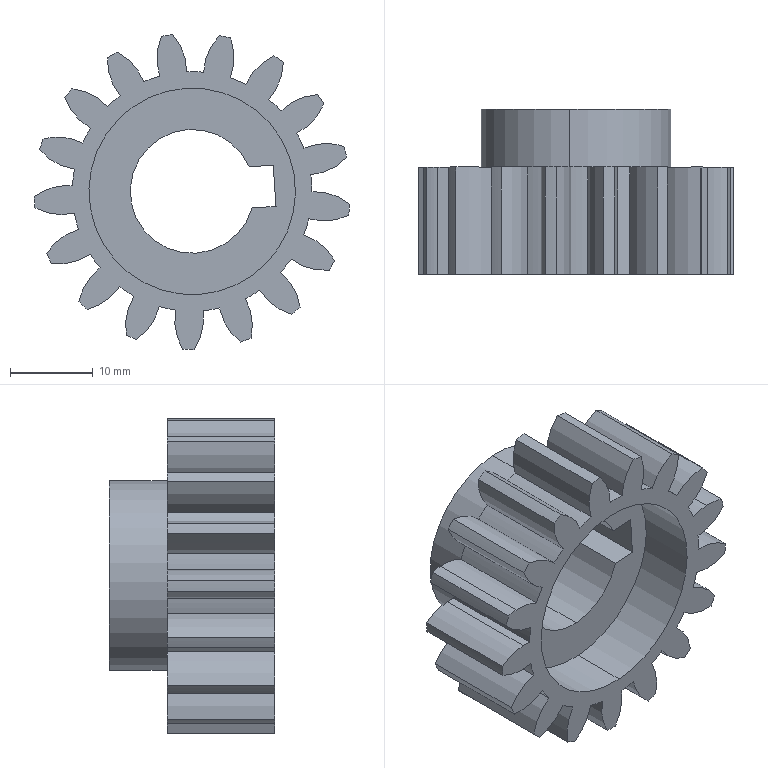Component | SolidWorks | GenevaWheelUpperGear(45Steel)-1 | 1 solid | 86 faces | box 38.22 x 20 x 38.14 mm | volume 8625 mm3 | cylinder 79 | plane 7 | commonest cylinder face diameters 13.6 x38 29 x17 38.289 x17 15 x3 25 x2 23 x2
build123d program:
from build123d import *

# Parameters (mm, degrees)
SKETCH1_R           = 14.5
BOSS_EXTRUDE1_DEPTH = 20
BOSS_EXTRUDE2_START = -13
BOSS_EXTRUDE2_DEPTH = 13
SKETCH4_R           = 14.5
SKETCH4_R_2         = 11.5
CUT_EXTRUDE1_DEPTH  = 7
CIRPATTERN1_COUNT   = 17
SKETCH5_R           = 12.5
CUT_EXTRUDE2_DEPTH  = 7


with BuildPart() as part:
    # Sketch1 → Boss-Extrude1 (new body)
    with BuildSketch(Plane.XY):
        Circle(SKETCH1_R)
        with BuildLine():
            Line((-2.5, -10), (2.5, -10))
            Line((2.5, -10), (2.5, -7.071))
            ThreePointArc((2.5, -7.071), (0, 7.5), (-2.5, -7.071))
            Line((-2.5, -7.071), (-2.5, -10))
        make_face(mode=Mode.SUBTRACT)
    extrude(amount=BOSS_EXTRUDE1_DEPTH)

    # Sketch3 → Boss-Extrude2 (add)
    with BuildSketch(Plane.XY.offset(20).offset(BOSS_EXTRUDE2_START)):
        with BuildLine():
            ThreePointArc((0.6859, 19.132), (0, 19.144), (-0.6859, 19.132))
            ThreePointArc((-0.6859, 19.132), (-1.604, 16.857), (-1.655, 14.405))
            ThreePointArc((-1.655, 14.405), (0, 14.5), (1.655, 14.405))
            ThreePointArc((1.655, 14.405), (1.604, 16.857), (0.6859, 19.132))
        make_face()
    boss_extrude2 = extrude(amount=BOSS_EXTRUDE2_DEPTH)

    # Sketch4 → Cut-Extrude1 (cut)
    with BuildSketch(Plane(origin=(0, 0, 0), x_dir=(-1, 0, 0), z_dir=(0, 0, -1))):
        Circle(SKETCH4_R)
        Circle(SKETCH4_R_2, mode=Mode.SUBTRACT)
    extrude(amount=-CUT_EXTRUDE1_DEPTH, mode=Mode.SUBTRACT)

    # CirPattern1: Boss-Extrude2 ×17 about axis
    cirpattern1_axis = Axis((0, 0, 0), (0, 0, 1))
    for i in range(1, CIRPATTERN1_COUNT):
        add(boss_extrude2.rotate(cirpattern1_axis, i * 360 / CIRPATTERN1_COUNT))

    # Sketch5 → Cut-Extrude2 (cut)
    with BuildSketch(Plane.XY.offset(20)):
        Circle(SKETCH5_R)
    extrude(amount=-CUT_EXTRUDE2_DEPTH, mode=Mode.SUBTRACT)


solid = part.part

# Placed as in the assembly
solid = solid.moved(Location((-27.344, 74.266, -166.507), (90, 0, 93.907)))